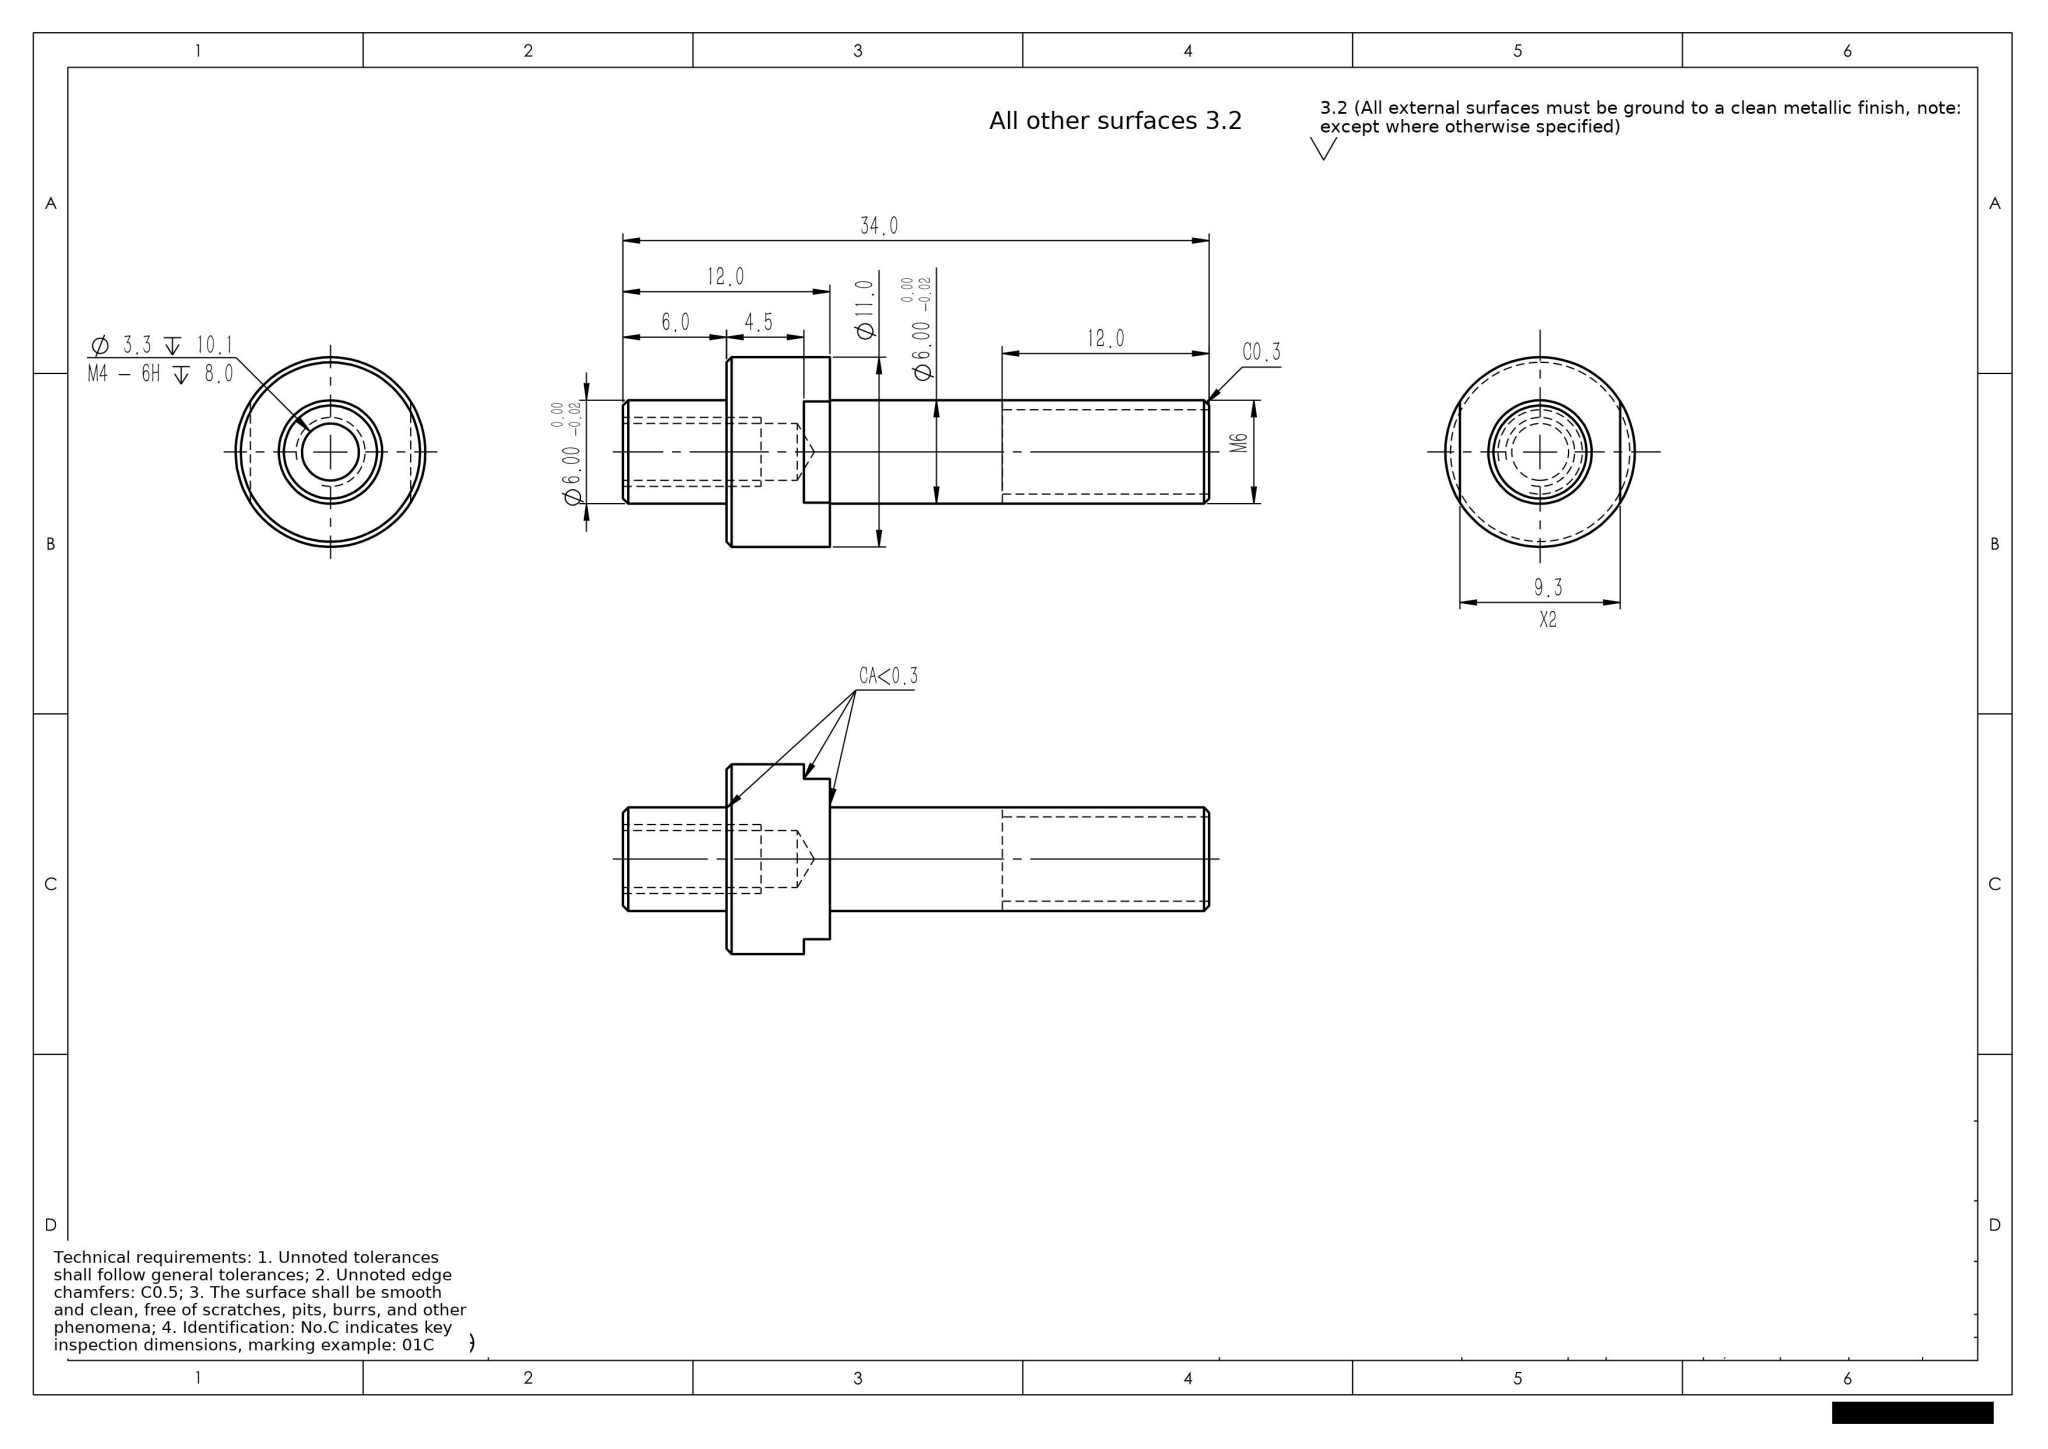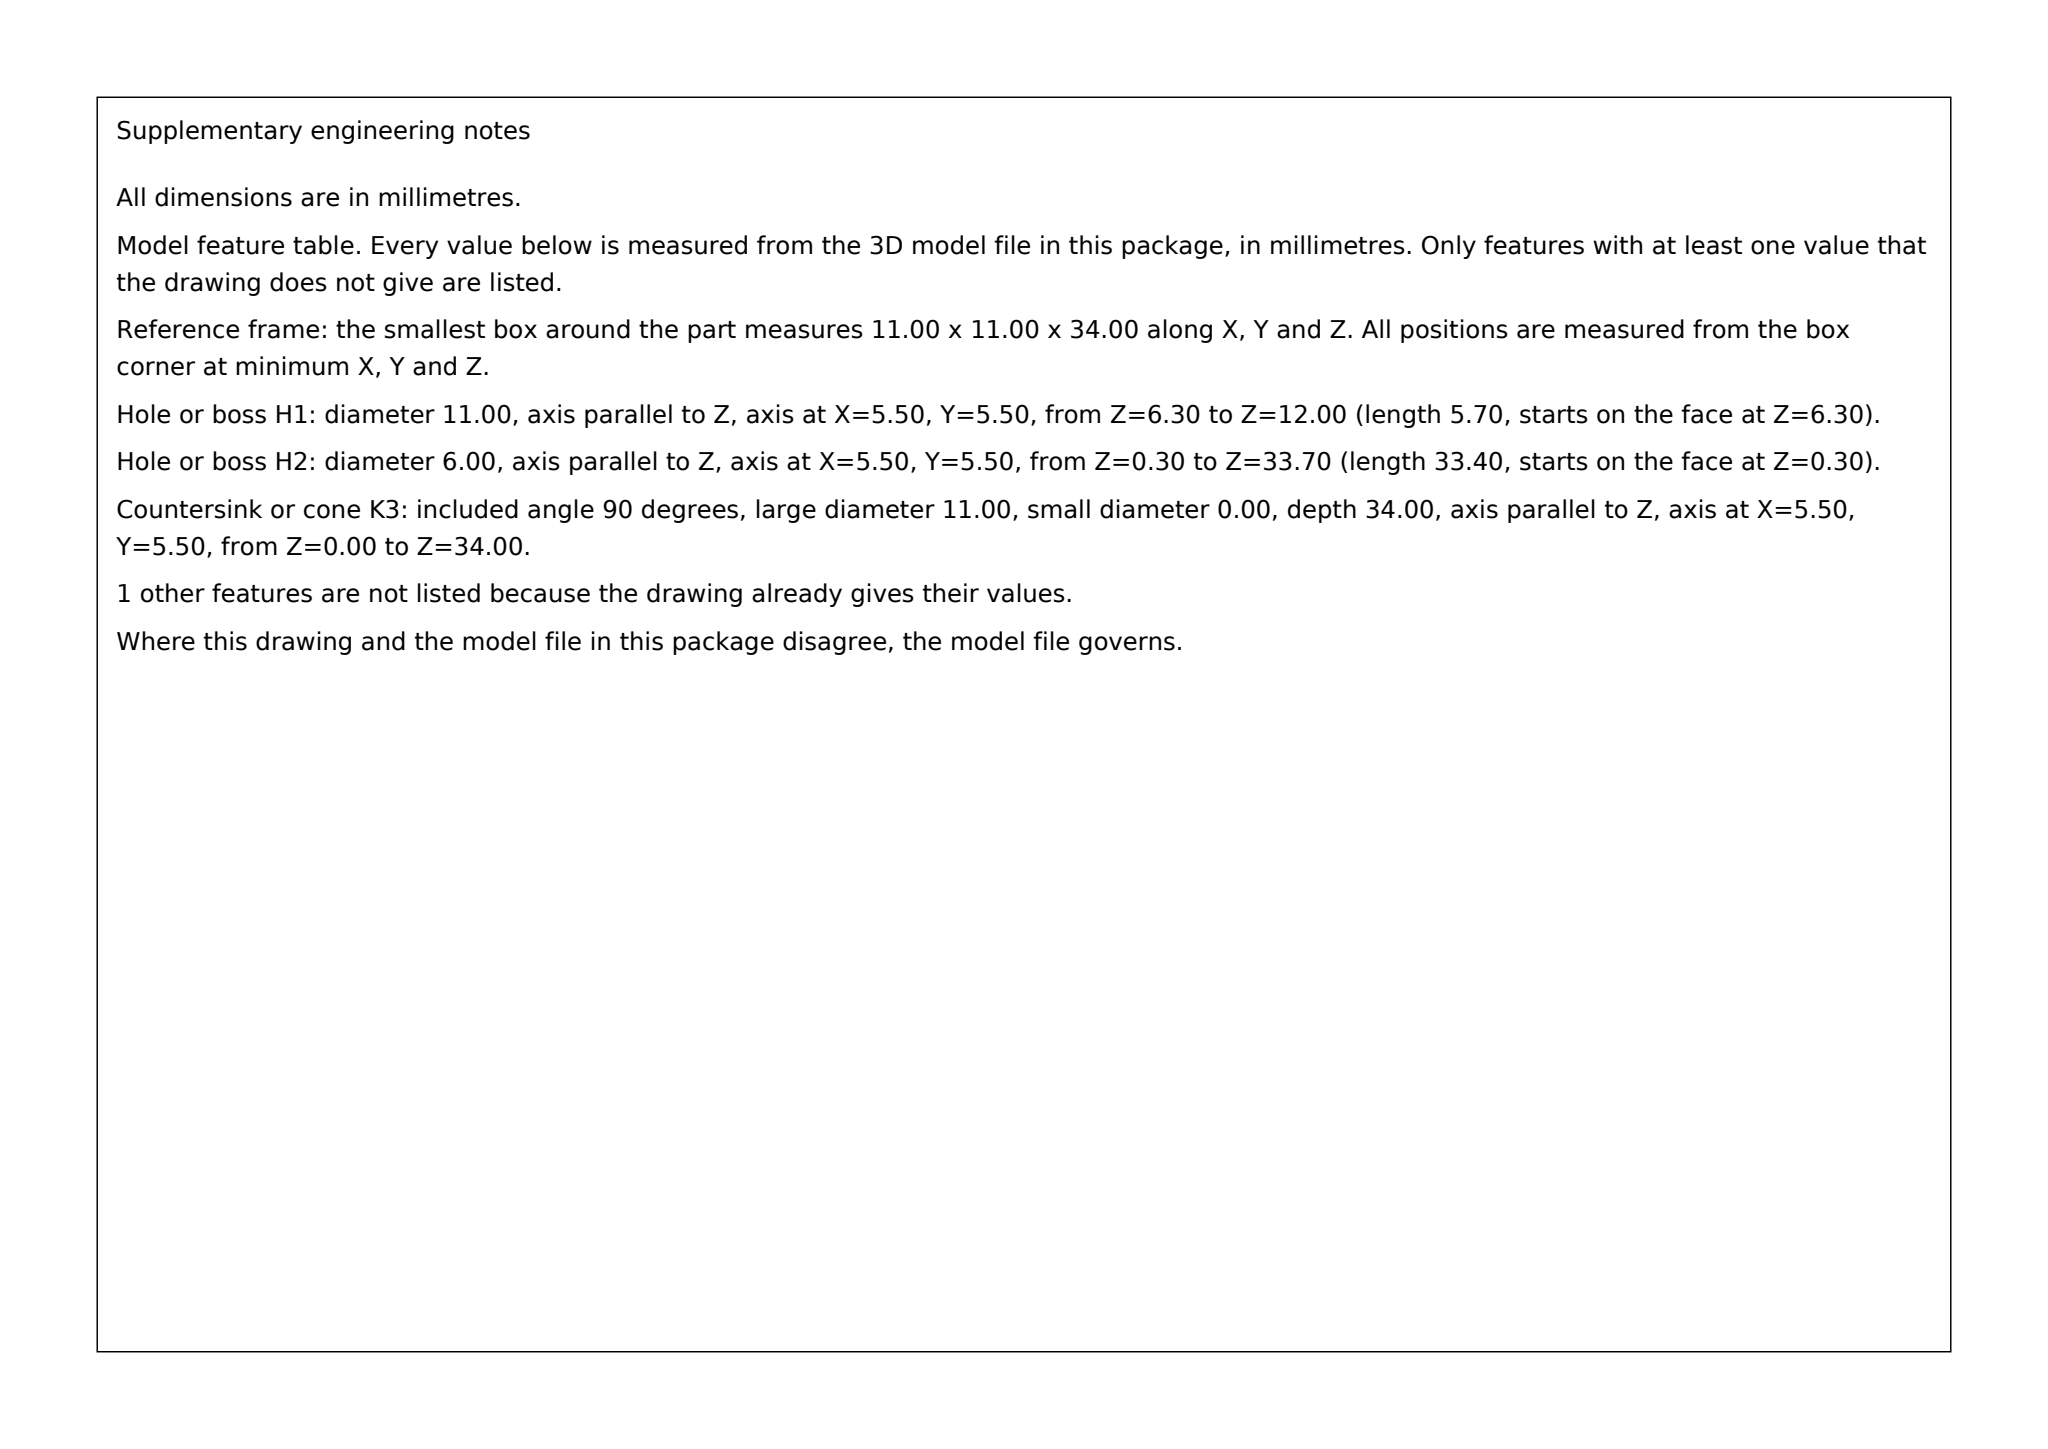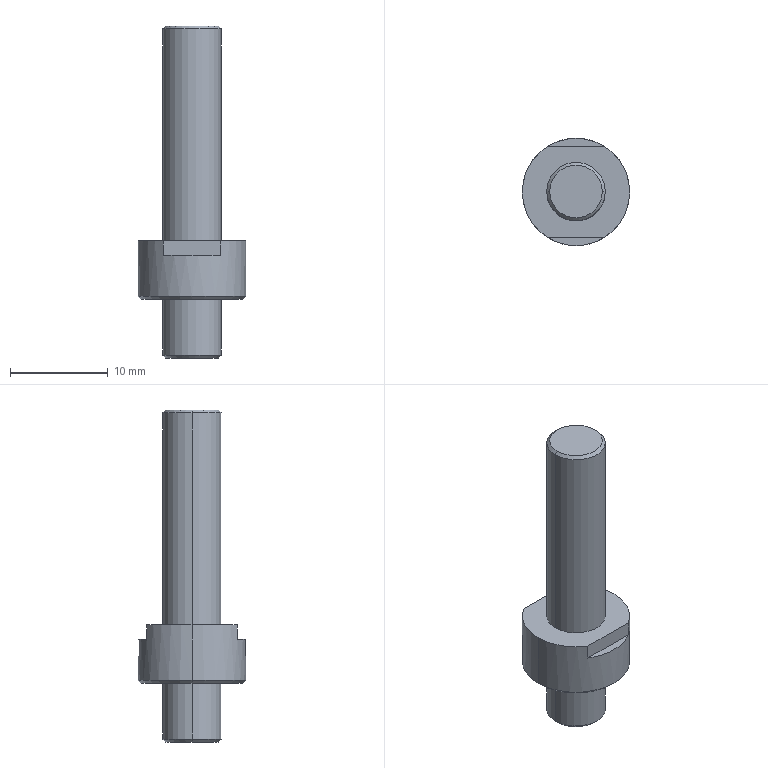Part | SolidWorks | mm | 1 solid | 24 faces | box 11 x 11 x 34 mm | volume 1259 mm3 | cone 8 | cylinder 8 | plane 8 | commonest cylinder face diameters 6 x4 3.3 x2 11 x2
build123d program:
from build123d import *

# Parameters (mm, degrees)
SKETCH1_R             = 5.5
BOSS_EXTRUDE1_DEPTH   = 6
SKETCH2_R             = 3
BOSS_EXTRUDE2_DEPTH   = 28
BOSS_EXTRUDE4_START   = 6
SKETCH3_R             = 3
BOSS_EXTRUDE4_DEPTH   = 6
M4_TAPPED_HOLE1_D     = 3.3
M4_TAPPED_HOLE1_DEPTH = 10.1
M4_TAPPED_HOLE1_TIP   = 0.9914
SKETCH6_OUTSIDE_W     = 20.478
SKETCH6_OUTSIDE_H     = 20.478
SKETCH6_OUTSIDE_W_2   = 12
SKETCH6_OUTSIDE_H_2   = 9.3
CUT_EXTRUDE1_DEPTH    = 1.5
CHAMFER1_SIZE         = 0.3


with BuildPart() as part:
    # Sketch1 → Boss-Extrude1 (new body)
    with BuildSketch(Plane.XY):
        Circle(SKETCH1_R)
    extrude(amount=BOSS_EXTRUDE1_DEPTH)

    # Sketch2 → Boss-Extrude2 (add)
    with BuildSketch(Plane.XY):
        Circle(SKETCH2_R)
    extrude(amount=BOSS_EXTRUDE2_DEPTH)

    # Sketch3 → Boss-Extrude4 (add)
    with BuildSketch(Plane(origin=(0, 0, 0), x_dir=(-1, 0, 0), z_dir=(0, 0, -1)).offset(BOSS_EXTRUDE4_START)):
        with Locations(Location((0, 0, 0), (0, 0, 180))):
            Circle(SKETCH3_R)
    extrude(amount=-BOSS_EXTRUDE4_DEPTH)

    # M4 Tapped Hole1
    with Locations(Plane(origin=(0, 0, -6), x_dir=(-1, 0, 0), z_dir=(0, 0, -1))):
        with Locations((0, 0)):
            Hole(M4_TAPPED_HOLE1_D / 2, depth=M4_TAPPED_HOLE1_DEPTH)
            with Locations((0, 0, -(M4_TAPPED_HOLE1_DEPTH + M4_TAPPED_HOLE1_TIP / 2))):  # 118° drill point
                Cone(0, M4_TAPPED_HOLE1_D / 2, M4_TAPPED_HOLE1_TIP, mode=Mode.SUBTRACT)

    # Sketch6 outside → Cut-Extrude1 (cut)
    with BuildSketch(Plane.XY.offset(6)):
        Rectangle(SKETCH6_OUTSIDE_W, SKETCH6_OUTSIDE_H)
        Rectangle(SKETCH6_OUTSIDE_W_2, SKETCH6_OUTSIDE_H_2, mode=Mode.SUBTRACT)
    extrude(amount=-CUT_EXTRUDE1_DEPTH, mode=Mode.SUBTRACT)

    # Chamfer1
    chamfer1_edges = [part.edges().sort_by_distance(p)[0] for p in [
        (-3, 0, -6),
        (-5.5, 0, 0),
        (-3, 0, 28),
    ]]
    chamfer(chamfer1_edges, length=CHAMFER1_SIZE)


solid = part.part
STEP:
#1=CARTESIAN_POINT('',(2.7,0.,28.));
#2=VERTEX_POINT('',#1);
#3=CARTESIAN_POINT('',(-2.7,0.,28.));
#4=VERTEX_POINT('',#3);
#5=CARTESIAN_POINT('',(0.,0.,28.));
#6=DIRECTION('',(0.,0.,1.));
#7=DIRECTION('',(1.,0.,0.));
#8=AXIS2_PLACEMENT_3D('',#5,#6,#7);
#9=CIRCLE('',#8,2.7);
#10=EDGE_CURVE('',#2,#4,#9,.T.);
#11=ORIENTED_EDGE('',*,*,#10,.F.);
#12=CARTESIAN_POINT('',(3.,0.,27.7));
#13=VERTEX_POINT('',#12);
#14=CARTESIAN_POINT('',(2.7,0.,28.));
#15=DIRECTION('',(0.7071,0.,-0.7071));
#16=VECTOR('',#15,1000.);
#17=LINE('',#14,#16);
#18=EDGE_CURVE('',#2,#13,#17,.T.);
#19=ORIENTED_EDGE('',*,*,#18,.T.);
#20=CARTESIAN_POINT('',(-3.,0.,27.7));
#21=VERTEX_POINT('',#20);
#22=CARTESIAN_POINT('',(0.,0.,27.7));
#23=DIRECTION('',(0.,0.,-1.));
#24=DIRECTION('',(1.,0.,0.));
#25=AXIS2_PLACEMENT_3D('',#22,#23,#24);
#26=CIRCLE('',#25,3.);
#27=EDGE_CURVE('',#21,#13,#26,.T.);
#28=ORIENTED_EDGE('',*,*,#27,.F.);
#29=CARTESIAN_POINT('',(-2.7,0.,28.));
#30=DIRECTION('',(-0.7071,0.,-0.7071));
#31=VECTOR('',#30,1000.);
#32=LINE('',#29,#31);
#33=EDGE_CURVE('',#4,#21,#32,.T.);
#34=ORIENTED_EDGE('',*,*,#33,.F.);
#35=EDGE_LOOP('',(#11,#19,#28,#34));
#36=FACE_OUTER_BOUND('',#35,.T.);
#37=CARTESIAN_POINT('',(0.,0.,28.));
#38=DIRECTION('',(0.,0.,-1.));
#39=DIRECTION('',(-1.,0.,0.));
#40=AXIS2_PLACEMENT_3D('',#37,#38,#39);
#41=CONICAL_SURFACE('',#40,2.7,0.7854);
#42=ADVANCED_FACE('',(#36),#41,.T.);
#43=CARTESIAN_POINT('',(-5.2,0.,0.));
#44=VERTEX_POINT('',#43);
#45=CARTESIAN_POINT('',(5.2,0.,0.));
#46=VERTEX_POINT('',#45);
#47=CARTESIAN_POINT('',(0.,0.,0.));
#48=DIRECTION('',(0.,0.,-1.));
#49=DIRECTION('',(1.,0.,0.));
#50=AXIS2_PLACEMENT_3D('',#47,#48,#49);
#51=CIRCLE('',#50,5.2);
#52=EDGE_CURVE('',#44,#46,#51,.T.);
#53=ORIENTED_EDGE('',*,*,#52,.F.);
#54=CARTESIAN_POINT('',(-5.5,0.,0.3));
#55=VERTEX_POINT('',#54);
#56=CARTESIAN_POINT('',(-5.5,0.,0.3));
#57=DIRECTION('',(-0.7071,0.,0.7071));
#58=VECTOR('',#57,1000.);
#59=LINE('',#56,#58);
#60=EDGE_CURVE('',#44,#55,#59,.T.);
#61=ORIENTED_EDGE('',*,*,#60,.T.);
#62=CARTESIAN_POINT('',(5.5,0.,0.3));
#63=VERTEX_POINT('',#62);
#64=CARTESIAN_POINT('',(0.,0.,0.3));
#65=DIRECTION('',(0.,0.,1.));
#66=DIRECTION('',(1.,0.,0.));
#67=AXIS2_PLACEMENT_3D('',#64,#65,#66);
#68=CIRCLE('',#67,5.5);
#69=EDGE_CURVE('',#63,#55,#68,.T.);
#70=ORIENTED_EDGE('',*,*,#69,.F.);
#71=CARTESIAN_POINT('',(5.5,0.,0.3));
#72=DIRECTION('',(0.7071,0.,0.7071));
#73=VECTOR('',#72,1000.);
#74=LINE('',#71,#73);
#75=EDGE_CURVE('',#46,#63,#74,.T.);
#76=ORIENTED_EDGE('',*,*,#75,.F.);
#77=EDGE_LOOP('',(#53,#61,#70,#76));
#78=FACE_OUTER_BOUND('',#77,.T.);
#79=CARTESIAN_POINT('',(0.,0.,0.3));
#80=DIRECTION('',(0.,0.,1.));
#81=DIRECTION('',(1.,0.,0.));
#82=AXIS2_PLACEMENT_3D('',#79,#80,#81);
#83=CONICAL_SURFACE('',#82,5.5,0.7854);
#84=ADVANCED_FACE('',(#78),#83,.T.);
#85=CARTESIAN_POINT('',(-2.7,0.,-6.));
#86=VERTEX_POINT('',#85);
#87=CARTESIAN_POINT('',(2.7,0.,-6.));
#88=VERTEX_POINT('',#87);
#89=CARTESIAN_POINT('',(0.,0.,-6.));
#90=DIRECTION('',(0.,0.,-1.));
#91=DIRECTION('',(-1.,0.,0.));
#92=AXIS2_PLACEMENT_3D('',#89,#90,#91);
#93=CIRCLE('',#92,2.7);
#94=EDGE_CURVE('',#86,#88,#93,.T.);
#95=ORIENTED_EDGE('',*,*,#94,.F.);
#96=CARTESIAN_POINT('',(-3.,0.,-5.7));
#97=VERTEX_POINT('',#96);
#98=CARTESIAN_POINT('',(-2.7,0.,-6.));
#99=DIRECTION('',(-0.7071,0.,0.7071));
#100=VECTOR('',#99,1000.);
#101=LINE('',#98,#100);
#102=EDGE_CURVE('',#86,#97,#101,.T.);
#103=ORIENTED_EDGE('',*,*,#102,.T.);
#104=CARTESIAN_POINT('',(3.,0.,-5.7));
#105=VERTEX_POINT('',#104);
#106=CARTESIAN_POINT('',(0.,0.,-5.7));
#107=DIRECTION('',(0.,0.,1.));
#108=DIRECTION('',(-1.,0.,0.));
#109=AXIS2_PLACEMENT_3D('',#106,#107,#108);
#110=CIRCLE('',#109,3.);
#111=EDGE_CURVE('',#105,#97,#110,.T.);
#112=ORIENTED_EDGE('',*,*,#111,.F.);
#113=CARTESIAN_POINT('',(2.7,0.,-6.));
#114=DIRECTION('',(0.7071,0.,0.7071));
#115=VECTOR('',#114,1000.);
#116=LINE('',#113,#115);
#117=EDGE_CURVE('',#88,#105,#116,.T.);
#118=ORIENTED_EDGE('',*,*,#117,.F.);
#119=EDGE_LOOP('',(#95,#103,#112,#118));
#120=FACE_OUTER_BOUND('',#119,.T.);
#121=CARTESIAN_POINT('',(0.,0.,-6.));
#122=DIRECTION('',(0.,0.,1.));
#123=DIRECTION('',(1.,0.,0.));
#124=AXIS2_PLACEMENT_3D('',#121,#122,#123);
#125=CONICAL_SURFACE('',#124,2.7,0.7854);
#126=ADVANCED_FACE('',(#120),#125,.T.);
#127=CARTESIAN_POINT('',(1.65,0.,4.1));
#128=VERTEX_POINT('',#127);
#129=CARTESIAN_POINT('',(-1.65,0.,4.1));
#130=VERTEX_POINT('',#129);
#131=CARTESIAN_POINT('',(0.,0.,4.1));
#132=DIRECTION('',(0.,0.,-1.));
#133=DIRECTION('',(-1.,0.,0.));
#134=AXIS2_PLACEMENT_3D('',#131,#132,#133);
#135=CIRCLE('',#134,1.65);
#136=EDGE_CURVE('',#128,#130,#135,.T.);
#137=ORIENTED_EDGE('',*,*,#136,.F.);
#138=CARTESIAN_POINT('',(1.65,0.,-6.));
#139=VERTEX_POINT('',#138);
#140=CARTESIAN_POINT('',(1.65,0.,-6.));
#141=DIRECTION('',(0.,0.,-1.));
#142=VECTOR('',#141,1000.);
#143=LINE('',#140,#142);
#144=EDGE_CURVE('',#128,#139,#143,.T.);
#145=ORIENTED_EDGE('',*,*,#144,.T.);
#146=CARTESIAN_POINT('',(-1.65,0.,-6.));
#147=VERTEX_POINT('',#146);
#148=CARTESIAN_POINT('',(0.,0.,-6.));
#149=DIRECTION('',(0.,0.,-1.));
#150=DIRECTION('',(-1.,0.,0.));
#151=AXIS2_PLACEMENT_3D('',#148,#149,#150);
#152=CIRCLE('',#151,1.65);
#153=EDGE_CURVE('',#139,#147,#152,.T.);
#154=ORIENTED_EDGE('',*,*,#153,.T.);
#155=CARTESIAN_POINT('',(-1.65,0.,-6.));
#156=DIRECTION('',(0.,0.,-1.));
#157=VECTOR('',#156,1000.);
#158=LINE('',#155,#157);
#159=EDGE_CURVE('',#130,#147,#158,.T.);
#160=ORIENTED_EDGE('',*,*,#159,.F.);
#161=EDGE_LOOP('',(#137,#145,#154,#160));
#162=FACE_OUTER_BOUND('',#161,.T.);
#163=CARTESIAN_POINT('',(0.,0.,-6.));
#164=DIRECTION('',(0.,0.,-1.));
#165=DIRECTION('',(-1.,0.,0.));
#166=AXIS2_PLACEMENT_3D('',#163,#164,#165);
#167=CYLINDRICAL_SURFACE('',#166,1.65);
#168=ADVANCED_FACE('',(#162),#167,.F.);
#169=CARTESIAN_POINT('',(-0.,0.,5.091));
#170=VERTEX_POINT('',#169);
#171=CARTESIAN_POINT('',(-1.65,0.,4.1));
#172=DIRECTION('',(-0.8572,0.,-0.515));
#173=VECTOR('',#172,1000.);
#174=LINE('',#171,#173);
#175=EDGE_CURVE('',#170,#130,#174,.T.);
#176=ORIENTED_EDGE('',*,*,#175,.F.);
#177=CARTESIAN_POINT('',(1.65,0.,4.1));
#178=DIRECTION('',(0.8572,0.,-0.515));
#179=VECTOR('',#178,1000.);
#180=LINE('',#177,#179);
#181=EDGE_CURVE('',#170,#128,#180,.T.);
#182=ORIENTED_EDGE('',*,*,#181,.T.);
#183=ORIENTED_EDGE('',*,*,#136,.T.);
#184=EDGE_LOOP('',(#176,#182,#183));
#185=FACE_OUTER_BOUND('',#184,.T.);
#186=CARTESIAN_POINT('',(0.,0.,4.1));
#187=DIRECTION('',(0.,0.,-1.));
#188=DIRECTION('',(-1.,0.,0.));
#189=AXIS2_PLACEMENT_3D('',#186,#187,#188);
#190=CONICAL_SURFACE('',#189,1.65,1.03);
#191=ADVANCED_FACE('',(#185),#190,.F.);
#192=ORIENTED_EDGE('',*,*,#111,.T.);
#193=CARTESIAN_POINT('',(-3.,0.,0.));
#194=VERTEX_POINT('',#193);
#195=CARTESIAN_POINT('',(-3.,0.,-6.));
#196=DIRECTION('',(0.,0.,1.));
#197=VECTOR('',#196,1000.);
#198=LINE('',#195,#197);
#199=EDGE_CURVE('',#97,#194,#198,.T.);
#200=ORIENTED_EDGE('',*,*,#199,.T.);
#201=CARTESIAN_POINT('',(3.,0.,0.));
#202=VERTEX_POINT('',#201);
#203=CARTESIAN_POINT('',(0.,0.,0.));
#204=DIRECTION('',(0.,0.,-1.));
#205=DIRECTION('',(1.,0.,0.));
#206=AXIS2_PLACEMENT_3D('',#203,#204,#205);
#207=CIRCLE('',#206,3.);
#208=EDGE_CURVE('',#194,#202,#207,.T.);
#209=ORIENTED_EDGE('',*,*,#208,.T.);
#210=CARTESIAN_POINT('',(3.,0.,-6.));
#211=DIRECTION('',(0.,0.,1.));
#212=VECTOR('',#211,1000.);
#213=LINE('',#210,#212);
#214=EDGE_CURVE('',#105,#202,#213,.T.);
#215=ORIENTED_EDGE('',*,*,#214,.F.);
#216=EDGE_LOOP('',(#192,#200,#209,#215));
#217=FACE_OUTER_BOUND('',#216,.T.);
#218=CARTESIAN_POINT('',(0.,0.,-6.));
#219=DIRECTION('',(0.,0.,1.));
#220=DIRECTION('',(1.,0.,0.));
#221=AXIS2_PLACEMENT_3D('',#218,#219,#220);
#222=CYLINDRICAL_SURFACE('',#221,3.);
#223=ADVANCED_FACE('',(#217),#222,.T.);
#224=ORIENTED_EDGE('',*,*,#27,.T.);
#225=CARTESIAN_POINT('',(3.,0.,6.));
#226=VERTEX_POINT('',#225);
#227=CARTESIAN_POINT('',(3.,0.,28.));
#228=DIRECTION('',(0.,0.,-1.));
#229=VECTOR('',#228,1000.);
#230=LINE('',#227,#229);
#231=EDGE_CURVE('',#13,#226,#230,.T.);
#232=ORIENTED_EDGE('',*,*,#231,.T.);
#233=CARTESIAN_POINT('',(-3.,0.,6.));
#234=VERTEX_POINT('',#233);
#235=CARTESIAN_POINT('',(0.,0.,6.));
#236=DIRECTION('',(0.,0.,-1.));
#237=DIRECTION('',(1.,0.,0.));
#238=AXIS2_PLACEMENT_3D('',#235,#236,#237);
#239=CIRCLE('',#238,3.);
#240=EDGE_CURVE('',#234,#226,#239,.T.);
#241=ORIENTED_EDGE('',*,*,#240,.F.);
#242=CARTESIAN_POINT('',(-3.,0.,28.));
#243=DIRECTION('',(0.,0.,-1.));
#244=VECTOR('',#243,1000.);
#245=LINE('',#242,#244);
#246=EDGE_CURVE('',#21,#234,#245,.T.);
#247=ORIENTED_EDGE('',*,*,#246,.F.);
#248=EDGE_LOOP('',(#224,#232,#241,#247));
#249=FACE_OUTER_BOUND('',#248,.T.);
#250=CARTESIAN_POINT('',(0.,0.,28.));
#251=DIRECTION('',(0.,0.,-1.));
#252=DIRECTION('',(-1.,0.,0.));
#253=AXIS2_PLACEMENT_3D('',#250,#251,#252);
#254=CYLINDRICAL_SURFACE('',#253,3.);
#255=ADVANCED_FACE('',(#249),#254,.T.);
#256=CARTESIAN_POINT('',(5.5,0.,6.));
#257=VERTEX_POINT('',#256);
#258=CARTESIAN_POINT('',(2.937,4.65,6.));
#259=VERTEX_POINT('',#258);
#260=CARTESIAN_POINT('',(0.,0.,6.));
#261=DIRECTION('',(0.,0.,1.));
#262=DIRECTION('',(1.,0.,0.));
#263=AXIS2_PLACEMENT_3D('',#260,#261,#262);
#264=CIRCLE('',#263,5.5);
#265=EDGE_CURVE('',#257,#259,#264,.T.);
#266=ORIENTED_EDGE('',*,*,#265,.F.);
#267=CARTESIAN_POINT('',(5.5,0.,6.));
#268=DIRECTION('',(0.,0.,-1.));
#269=VECTOR('',#268,1000.);
#270=LINE('',#267,#269);
#271=EDGE_CURVE('',#257,#63,#270,.T.);
#272=ORIENTED_EDGE('',*,*,#271,.T.);
#273=ORIENTED_EDGE('',*,*,#69,.T.);
#274=CARTESIAN_POINT('',(-5.5,0.,6.));
#275=VERTEX_POINT('',#274);
#276=CARTESIAN_POINT('',(-5.5,0.,6.));
#277=DIRECTION('',(0.,0.,-1.));
#278=VECTOR('',#277,1000.);
#279=LINE('',#276,#278);
#280=EDGE_CURVE('',#275,#55,#279,.T.);
#281=ORIENTED_EDGE('',*,*,#280,.F.);
#282=CARTESIAN_POINT('',(-2.937,4.65,6.));
#283=VERTEX_POINT('',#282);
#284=CARTESIAN_POINT('',(0.,0.,6.));
#285=DIRECTION('',(0.,0.,1.));
#286=DIRECTION('',(1.,0.,0.));
#287=AXIS2_PLACEMENT_3D('',#284,#285,#286);
#288=CIRCLE('',#287,5.5);
#289=EDGE_CURVE('',#283,#275,#288,.T.);
#290=ORIENTED_EDGE('',*,*,#289,.F.);
#291=CARTESIAN_POINT('',(-2.937,4.65,4.5));
#292=VERTEX_POINT('',#291);
#293=CARTESIAN_POINT('',(-2.937,4.65,6.));
#294=DIRECTION('',(0.,0.,1.));
#295=VECTOR('',#294,1000.);
#296=LINE('',#293,#295);
#297=EDGE_CURVE('',#292,#283,#296,.T.);
#298=ORIENTED_EDGE('',*,*,#297,.F.);
#299=CARTESIAN_POINT('',(2.937,4.65,4.5));
#300=VERTEX_POINT('',#299);
#301=CARTESIAN_POINT('',(0.,0.,4.5));
#302=DIRECTION('',(0.,0.,1.));
#303=DIRECTION('',(1.,0.,0.));
#304=AXIS2_PLACEMENT_3D('',#301,#302,#303);
#305=CIRCLE('',#304,5.5);
#306=EDGE_CURVE('',#300,#292,#305,.T.);
#307=ORIENTED_EDGE('',*,*,#306,.F.);
#308=CARTESIAN_POINT('',(2.937,4.65,6.));
#309=DIRECTION('',(0.,0.,-1.));
#310=VECTOR('',#309,1000.);
#311=LINE('',#308,#310);
#312=EDGE_CURVE('',#259,#300,#311,.T.);
#313=ORIENTED_EDGE('',*,*,#312,.F.);
#314=EDGE_LOOP('',(#266,#272,#273,#281,#290,#298,#307,#313));
#315=FACE_OUTER_BOUND('',#314,.T.);
#316=CARTESIAN_POINT('',(0.,0.,6.));
#317=DIRECTION('',(0.,0.,-1.));
#318=DIRECTION('',(-1.,0.,0.));
#319=AXIS2_PLACEMENT_3D('',#316,#317,#318);
#320=CYLINDRICAL_SURFACE('',#319,5.5);
#321=ADVANCED_FACE('',(#315),#320,.T.);
#322=ORIENTED_EDGE('',*,*,#240,.T.);
#323=CARTESIAN_POINT('',(0.,0.,6.));
#324=DIRECTION('',(0.,0.,-1.));
#325=DIRECTION('',(1.,0.,0.));
#326=AXIS2_PLACEMENT_3D('',#323,#324,#325);
#327=CIRCLE('',#326,3.);
#328=EDGE_CURVE('',#226,#234,#327,.T.);
#329=ORIENTED_EDGE('',*,*,#328,.T.);
#330=EDGE_LOOP('',(#322,#329));
#331=FACE_BOUND('',#330,.T.);
#332=ORIENTED_EDGE('',*,*,#289,.T.);
#333=CARTESIAN_POINT('',(-2.937,-4.65,6.));
#334=VERTEX_POINT('',#333);
#335=CARTESIAN_POINT('',(0.,0.,6.));
#336=DIRECTION('',(0.,0.,1.));
#337=DIRECTION('',(1.,0.,0.));
#338=AXIS2_PLACEMENT_3D('',#335,#336,#337);
#339=CIRCLE('',#338,5.5);
#340=EDGE_CURVE('',#275,#334,#339,.T.);
#341=ORIENTED_EDGE('',*,*,#340,.T.);
#342=CARTESIAN_POINT('',(2.937,-4.65,6.));
#343=VERTEX_POINT('',#342);
#344=CARTESIAN_POINT('',(-6.,-4.65,6.));
#345=DIRECTION('',(1.,0.,0.));
#346=VECTOR('',#345,1000.);
#347=LINE('',#344,#346);
#348=EDGE_CURVE('',#334,#343,#347,.T.);
#349=ORIENTED_EDGE('',*,*,#348,.T.);
#350=CARTESIAN_POINT('',(0.,0.,6.));
#351=DIRECTION('',(0.,0.,1.));
#352=DIRECTION('',(1.,0.,0.));
#353=AXIS2_PLACEMENT_3D('',#350,#351,#352);
#354=CIRCLE('',#353,5.5);
#355=EDGE_CURVE('',#343,#257,#354,.T.);
#356=ORIENTED_EDGE('',*,*,#355,.T.);
#357=ORIENTED_EDGE('',*,*,#265,.T.);
#358=CARTESIAN_POINT('',(-6.,4.65,6.));
#359=DIRECTION('',(-1.,0.,0.));
#360=VECTOR('',#359,1000.);
#361=LINE('',#358,#360);
#362=EDGE_CURVE('',#259,#283,#361,.T.);
#363=ORIENTED_EDGE('',*,*,#362,.T.);
#364=EDGE_LOOP('',(#332,#341,#349,#356,#357,#363));
#365=FACE_OUTER_BOUND('',#364,.T.);
#366=CARTESIAN_POINT('',(0.,0.,6.));
#367=DIRECTION('',(0.,0.,1.));
#368=DIRECTION('',(1.,0.,0.));
#369=AXIS2_PLACEMENT_3D('',#366,#367,#368);
#370=PLANE('',#369);
#371=ADVANCED_FACE('',(#331,#365),#370,.T.);
#372=ORIENTED_EDGE('',*,*,#271,.F.);
#373=ORIENTED_EDGE('',*,*,#355,.F.);
#374=CARTESIAN_POINT('',(2.937,-4.65,4.5));
#375=VERTEX_POINT('',#374);
#376=CARTESIAN_POINT('',(2.937,-4.65,6.));
#377=DIRECTION('',(0.,0.,1.));
#378=VECTOR('',#377,1000.);
#379=LINE('',#376,#378);
#380=EDGE_CURVE('',#375,#343,#379,.T.);
#381=ORIENTED_EDGE('',*,*,#380,.F.);
#382=CARTESIAN_POINT('',(-2.937,-4.65,4.5));
#383=VERTEX_POINT('',#382);
#384=CARTESIAN_POINT('',(0.,0.,4.5));
#385=DIRECTION('',(0.,0.,1.));
#386=DIRECTION('',(1.,0.,0.));
#387=AXIS2_PLACEMENT_3D('',#384,#385,#386);
#388=CIRCLE('',#387,5.5);
#389=EDGE_CURVE('',#383,#375,#388,.T.);
#390=ORIENTED_EDGE('',*,*,#389,.F.);
#391=CARTESIAN_POINT('',(-2.937,-4.65,6.));
#392=DIRECTION('',(0.,0.,-1.));
#393=VECTOR('',#392,1000.);
#394=LINE('',#391,#393);
#395=EDGE_CURVE('',#334,#383,#394,.T.);
#396=ORIENTED_EDGE('',*,*,#395,.F.);
#397=ORIENTED_EDGE('',*,*,#340,.F.);
#398=ORIENTED_EDGE('',*,*,#280,.T.);
#399=CARTESIAN_POINT('',(0.,0.,0.3));
#400=DIRECTION('',(0.,0.,1.));
#401=DIRECTION('',(1.,0.,0.));
#402=AXIS2_PLACEMENT_3D('',#399,#400,#401);
#403=CIRCLE('',#402,5.5);
#404=EDGE_CURVE('',#55,#63,#403,.T.);
#405=ORIENTED_EDGE('',*,*,#404,.T.);
#406=EDGE_LOOP('',(#372,#373,#381,#390,#396,#397,#398,#405));
#407=FACE_OUTER_BOUND('',#406,.T.);
#408=CARTESIAN_POINT('',(0.,0.,6.));
#409=DIRECTION('',(0.,0.,-1.));
#410=DIRECTION('',(-1.,0.,0.));
#411=AXIS2_PLACEMENT_3D('',#408,#409,#410);
#412=CYLINDRICAL_SURFACE('',#411,5.5);
#413=ADVANCED_FACE('',(#407),#412,.T.);
#414=CARTESIAN_POINT('',(0.,0.,0.));
#415=DIRECTION('',(0.,0.,-1.));
#416=DIRECTION('',(1.,0.,0.));
#417=AXIS2_PLACEMENT_3D('',#414,#415,#416);
#418=CIRCLE('',#417,5.2);
#419=EDGE_CURVE('',#46,#44,#418,.T.);
#420=ORIENTED_EDGE('',*,*,#419,.T.);
#421=ORIENTED_EDGE('',*,*,#52,.T.);
#422=EDGE_LOOP('',(#420,#421));
#423=FACE_OUTER_BOUND('',#422,.T.);
#424=CARTESIAN_POINT('',(0.,0.,0.));
#425=DIRECTION('',(0.,0.,-1.));
#426=DIRECTION('',(1.,0.,0.));
#427=AXIS2_PLACEMENT_3D('',#424,#425,#426);
#428=CIRCLE('',#427,3.);
#429=EDGE_CURVE('',#202,#194,#428,.T.);
#430=ORIENTED_EDGE('',*,*,#429,.F.);
#431=ORIENTED_EDGE('',*,*,#208,.F.);
#432=EDGE_LOOP('',(#430,#431));
#433=FACE_BOUND('',#432,.T.);
#434=CARTESIAN_POINT('',(0.,0.,0.));
#435=DIRECTION('',(0.,0.,1.));
#436=DIRECTION('',(1.,0.,0.));
#437=AXIS2_PLACEMENT_3D('',#434,#435,#436);
#438=PLANE('',#437);
#439=ADVANCED_FACE('',(#423,#433),#438,.F.);
#440=ORIENTED_EDGE('',*,*,#231,.F.);
#441=CARTESIAN_POINT('',(0.,0.,27.7));
#442=DIRECTION('',(0.,0.,-1.));
#443=DIRECTION('',(1.,0.,0.));
#444=AXIS2_PLACEMENT_3D('',#441,#442,#443);
#445=CIRCLE('',#444,3.);
#446=EDGE_CURVE('',#13,#21,#445,.T.);
#447=ORIENTED_EDGE('',*,*,#446,.T.);
#448=ORIENTED_EDGE('',*,*,#246,.T.);
#449=ORIENTED_EDGE('',*,*,#328,.F.);
#450=EDGE_LOOP('',(#440,#447,#448,#449));
#451=FACE_OUTER_BOUND('',#450,.T.);
#452=CARTESIAN_POINT('',(0.,0.,28.));
#453=DIRECTION('',(0.,0.,-1.));
#454=DIRECTION('',(-1.,0.,0.));
#455=AXIS2_PLACEMENT_3D('',#452,#453,#454);
#456=CYLINDRICAL_SURFACE('',#455,3.);
#457=ADVANCED_FACE('',(#451),#456,.T.);
#458=CARTESIAN_POINT('',(0.,0.,28.));
#459=DIRECTION('',(0.,0.,1.));
#460=DIRECTION('',(1.,0.,0.));
#461=AXIS2_PLACEMENT_3D('',#458,#459,#460);
#462=CIRCLE('',#461,2.7);
#463=EDGE_CURVE('',#4,#2,#462,.T.);
#464=ORIENTED_EDGE('',*,*,#463,.T.);
#465=ORIENTED_EDGE('',*,*,#10,.T.);
#466=EDGE_LOOP('',(#464,#465));
#467=FACE_OUTER_BOUND('',#466,.T.);
#468=CARTESIAN_POINT('',(0.,0.,28.));
#469=DIRECTION('',(0.,0.,1.));
#470=DIRECTION('',(1.,0.,0.));
#471=AXIS2_PLACEMENT_3D('',#468,#469,#470);
#472=PLANE('',#471);
#473=ADVANCED_FACE('',(#467),#472,.T.);
#474=ORIENTED_EDGE('',*,*,#199,.F.);
#475=CARTESIAN_POINT('',(0.,0.,-5.7));
#476=DIRECTION('',(0.,0.,1.));
#477=DIRECTION('',(-1.,0.,0.));
#478=AXIS2_PLACEMENT_3D('',#475,#476,#477);
#479=CIRCLE('',#478,3.);
#480=EDGE_CURVE('',#97,#105,#479,.T.);
#481=ORIENTED_EDGE('',*,*,#480,.T.);
#482=ORIENTED_EDGE('',*,*,#214,.T.);
#483=ORIENTED_EDGE('',*,*,#429,.T.);
#484=EDGE_LOOP('',(#474,#481,#482,#483));
#485=FACE_OUTER_BOUND('',#484,.T.);
#486=CARTESIAN_POINT('',(0.,0.,-6.));
#487=DIRECTION('',(0.,0.,1.));
#488=DIRECTION('',(1.,0.,0.));
#489=AXIS2_PLACEMENT_3D('',#486,#487,#488);
#490=CYLINDRICAL_SURFACE('',#489,3.);
#491=ADVANCED_FACE('',(#485),#490,.T.);
#492=CARTESIAN_POINT('',(0.,0.,-6.));
#493=DIRECTION('',(0.,0.,-1.));
#494=DIRECTION('',(-1.,0.,0.));
#495=AXIS2_PLACEMENT_3D('',#492,#493,#494);
#496=CIRCLE('',#495,2.7);
#497=EDGE_CURVE('',#88,#86,#496,.T.);
#498=ORIENTED_EDGE('',*,*,#497,.T.);
#499=ORIENTED_EDGE('',*,*,#94,.T.);
#500=EDGE_LOOP('',(#498,#499));
#501=FACE_OUTER_BOUND('',#500,.T.);
#502=CARTESIAN_POINT('',(0.,0.,-6.));
#503=DIRECTION('',(0.,0.,-1.));
#504=DIRECTION('',(-1.,0.,0.));
#505=AXIS2_PLACEMENT_3D('',#502,#503,#504);
#506=CIRCLE('',#505,1.65);
#507=EDGE_CURVE('',#147,#139,#506,.T.);
#508=ORIENTED_EDGE('',*,*,#507,.F.);
#509=ORIENTED_EDGE('',*,*,#153,.F.);
#510=EDGE_LOOP('',(#508,#509));
#511=FACE_BOUND('',#510,.T.);
#512=CARTESIAN_POINT('',(0.,0.,-6.));
#513=DIRECTION('',(0.,0.,-1.));
#514=DIRECTION('',(-1.,0.,0.));
#515=AXIS2_PLACEMENT_3D('',#512,#513,#514);
#516=PLANE('',#515);
#517=ADVANCED_FACE('',(#501,#511),#516,.T.);
#518=ORIENTED_EDGE('',*,*,#181,.F.);
#519=ORIENTED_EDGE('',*,*,#175,.T.);
#520=CARTESIAN_POINT('',(0.,0.,4.1));
#521=DIRECTION('',(0.,0.,-1.));
#522=DIRECTION('',(-1.,0.,0.));
#523=AXIS2_PLACEMENT_3D('',#520,#521,#522);
#524=CIRCLE('',#523,1.65);
#525=EDGE_CURVE('',#130,#128,#524,.T.);
#526=ORIENTED_EDGE('',*,*,#525,.T.);
#527=EDGE_LOOP('',(#518,#519,#526));
#528=FACE_OUTER_BOUND('',#527,.T.);
#529=CARTESIAN_POINT('',(0.,0.,4.1));
#530=DIRECTION('',(0.,0.,-1.));
#531=DIRECTION('',(-1.,0.,0.));
#532=AXIS2_PLACEMENT_3D('',#529,#530,#531);
#533=CONICAL_SURFACE('',#532,1.65,1.03);
#534=ADVANCED_FACE('',(#528),#533,.F.);
#535=ORIENTED_EDGE('',*,*,#144,.F.);
#536=ORIENTED_EDGE('',*,*,#525,.F.);
#537=ORIENTED_EDGE('',*,*,#159,.T.);
#538=ORIENTED_EDGE('',*,*,#507,.T.);
#539=EDGE_LOOP('',(#535,#536,#537,#538));
#540=FACE_OUTER_BOUND('',#539,.T.);
#541=CARTESIAN_POINT('',(0.,0.,-6.));
#542=DIRECTION('',(0.,0.,-1.));
#543=DIRECTION('',(-1.,0.,0.));
#544=AXIS2_PLACEMENT_3D('',#541,#542,#543);
#545=CYLINDRICAL_SURFACE('',#544,1.65);
#546=ADVANCED_FACE('',(#540),#545,.F.);
#547=ORIENTED_EDGE('',*,*,#312,.T.);
#548=CARTESIAN_POINT('',(-6.,4.65,4.5));
#549=DIRECTION('',(-1.,0.,0.));
#550=VECTOR('',#549,1000.);
#551=LINE('',#548,#550);
#552=EDGE_CURVE('',#300,#292,#551,.T.);
#553=ORIENTED_EDGE('',*,*,#552,.T.);
#554=ORIENTED_EDGE('',*,*,#297,.T.);
#555=ORIENTED_EDGE('',*,*,#362,.F.);
#556=EDGE_LOOP('',(#547,#553,#554,#555));
#557=FACE_OUTER_BOUND('',#556,.T.);
#558=CARTESIAN_POINT('',(-6.,4.65,4.5));
#559=DIRECTION('',(0.,1.,0.));
#560=DIRECTION('',(0.,0.,1.));
#561=AXIS2_PLACEMENT_3D('',#558,#559,#560);
#562=PLANE('',#561);
#563=ADVANCED_FACE('',(#557),#562,.T.);
#564=ORIENTED_EDGE('',*,*,#306,.T.);
#565=ORIENTED_EDGE('',*,*,#552,.F.);
#566=EDGE_LOOP('',(#564,#565));
#567=FACE_OUTER_BOUND('',#566,.T.);
#568=CARTESIAN_POINT('',(0.,0.,4.5));
#569=DIRECTION('',(0.,0.,1.));
#570=DIRECTION('',(1.,0.,0.));
#571=AXIS2_PLACEMENT_3D('',#568,#569,#570);
#572=PLANE('',#571);
#573=ADVANCED_FACE('',(#567),#572,.T.);
#574=ORIENTED_EDGE('',*,*,#389,.T.);
#575=CARTESIAN_POINT('',(-6.,-4.65,4.5));
#576=DIRECTION('',(1.,0.,0.));
#577=VECTOR('',#576,1000.);
#578=LINE('',#575,#577);
#579=EDGE_CURVE('',#383,#375,#578,.T.);
#580=ORIENTED_EDGE('',*,*,#579,.F.);
#581=EDGE_LOOP('',(#574,#580));
#582=FACE_OUTER_BOUND('',#581,.T.);
#583=CARTESIAN_POINT('',(0.,0.,4.5));
#584=DIRECTION('',(0.,0.,1.));
#585=DIRECTION('',(1.,0.,0.));
#586=AXIS2_PLACEMENT_3D('',#583,#584,#585);
#587=PLANE('',#586);
#588=ADVANCED_FACE('',(#582),#587,.T.);
#589=ORIENTED_EDGE('',*,*,#395,.T.);
#590=ORIENTED_EDGE('',*,*,#579,.T.);
#591=ORIENTED_EDGE('',*,*,#380,.T.);
#592=ORIENTED_EDGE('',*,*,#348,.F.);
#593=EDGE_LOOP('',(#589,#590,#591,#592));
#594=FACE_OUTER_BOUND('',#593,.T.);
#595=CARTESIAN_POINT('',(-6.,-4.65,4.5));
#596=DIRECTION('',(0.,-1.,0.));
#597=DIRECTION('',(0.,0.,-1.));
#598=AXIS2_PLACEMENT_3D('',#595,#596,#597);
#599=PLANE('',#598);
#600=ADVANCED_FACE('',(#594),#599,.T.);
#601=ORIENTED_EDGE('',*,*,#102,.F.);
#602=ORIENTED_EDGE('',*,*,#497,.F.);
#603=ORIENTED_EDGE('',*,*,#117,.T.);
#604=ORIENTED_EDGE('',*,*,#480,.F.);
#605=EDGE_LOOP('',(#601,#602,#603,#604));
#606=FACE_OUTER_BOUND('',#605,.T.);
#607=CARTESIAN_POINT('',(0.,0.,-6.));
#608=DIRECTION('',(0.,0.,1.));
#609=DIRECTION('',(1.,0.,0.));
#610=AXIS2_PLACEMENT_3D('',#607,#608,#609);
#611=CONICAL_SURFACE('',#610,2.7,0.7854);
#612=ADVANCED_FACE('',(#606),#611,.T.);
#613=ORIENTED_EDGE('',*,*,#60,.F.);
#614=ORIENTED_EDGE('',*,*,#419,.F.);
#615=ORIENTED_EDGE('',*,*,#75,.T.);
#616=ORIENTED_EDGE('',*,*,#404,.F.);
#617=EDGE_LOOP('',(#613,#614,#615,#616));
#618=FACE_OUTER_BOUND('',#617,.T.);
#619=CARTESIAN_POINT('',(0.,0.,0.3));
#620=DIRECTION('',(0.,0.,1.));
#621=DIRECTION('',(1.,0.,0.));
#622=AXIS2_PLACEMENT_3D('',#619,#620,#621);
#623=CONICAL_SURFACE('',#622,5.5,0.7854);
#624=ADVANCED_FACE('',(#618),#623,.T.);
#625=ORIENTED_EDGE('',*,*,#18,.F.);
#626=ORIENTED_EDGE('',*,*,#463,.F.);
#627=ORIENTED_EDGE('',*,*,#33,.T.);
#628=ORIENTED_EDGE('',*,*,#446,.F.);
#629=EDGE_LOOP('',(#625,#626,#627,#628));
#630=FACE_OUTER_BOUND('',#629,.T.);
#631=CARTESIAN_POINT('',(0.,0.,28.));
#632=DIRECTION('',(0.,0.,-1.));
#633=DIRECTION('',(-1.,0.,0.));
#634=AXIS2_PLACEMENT_3D('',#631,#632,#633);
#635=CONICAL_SURFACE('',#634,2.7,0.7854);
#636=ADVANCED_FACE('',(#630),#635,.T.);
#637=CLOSED_SHELL('',(#42,#84,#126,#168,#191,#223,#255,#321,#371,#413,#439,#457,#473,#491,#517,#534,#546,#563,#573,#588,#600,#612,#624,#636));
#638=MANIFOLD_SOLID_BREP('',#637);
#639=CARTESIAN_POINT('',(0.,0.,0.));
#640=DIRECTION('',(0.,0.,1.));
#641=DIRECTION('',(1.,0.,0.));
#642=AXIS2_PLACEMENT_3D('',#639,#640,#641);
#643=(LENGTH_UNIT()NAMED_UNIT(*)SI_UNIT(.MILLI.,.METRE.));
#644=UNCERTAINTY_MEASURE_WITH_UNIT(LENGTH_MEASURE(0.00001),#643,'','');
#645=(NAMED_UNIT(*)PLANE_ANGLE_UNIT()SI_UNIT($,.RADIAN.));
#646=(NAMED_UNIT(*)SI_UNIT($,.STERADIAN.)SOLID_ANGLE_UNIT());
#647=(GEOMETRIC_REPRESENTATION_CONTEXT(3)GLOBAL_UNCERTAINTY_ASSIGNED_CONTEXT((#644))GLOBAL_UNIT_ASSIGNED_CONTEXT((#643,#645,#646))REPRESENTATION_CONTEXT('',''));
#648=ADVANCED_BREP_SHAPE_REPRESENTATION('',(#638,#642),#647);